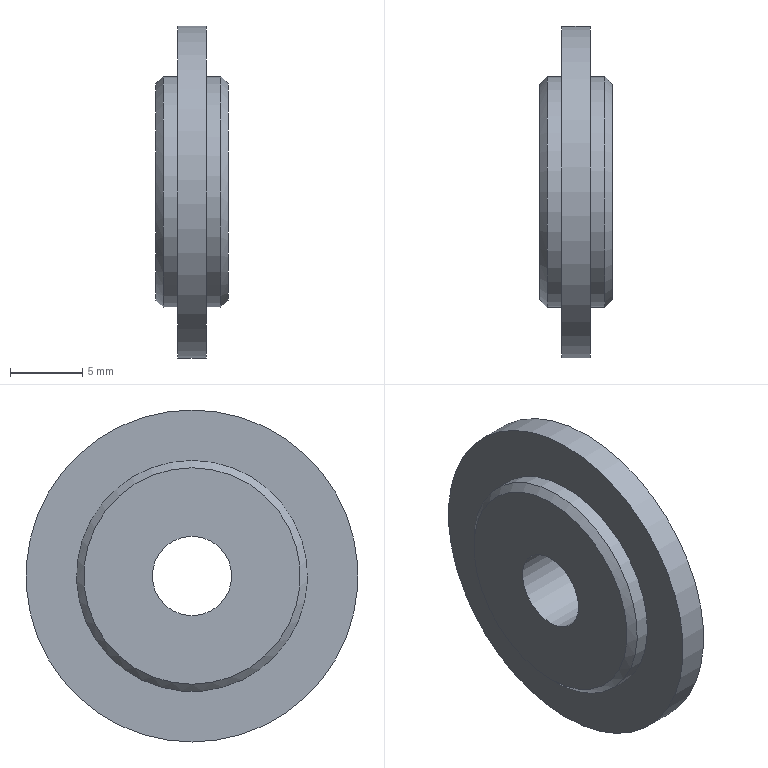Component | NX | MIDDLE_SPACER | 1 solid | 10 faces | box 5 x 23 x 23 mm | volume 1303 mm3 | cylinder 4 | plane 4 | cone 2 | commonest cylinder face diameters 16 x2 23 x1 5.5 x1
STEP:
#1=CARTESIAN_POINT('',(0.,0.,0.));
#2=DIRECTION('',(0.,0.,1.));
#3=DIRECTION('',(1.,0.,0.));
#4=AXIS2_PLACEMENT_3D('',#1,#2,#3);
#5=CARTESIAN_POINT('',(95.166,163.398,160.15));
#6=VERTEX_POINT('',#5);
#7=CARTESIAN_POINT('',(95.166,163.398,152.15));
#8=DIRECTION('',(-1.,0.,0.));
#9=DIRECTION('',(0.,0.,1.));
#10=AXIS2_PLACEMENT_3D('',#7,#8,#9);
#11=CIRCLE('',#10,8.);
#12=CARTESIAN_POINT('',(94.166,163.398,152.15));
#13=DIRECTION('',(1.,0.,0.));
#14=DIRECTION('',(0.,0.,-1.));
#15=AXIS2_PLACEMENT_3D('',#12,#13,#14);
#16=CYLINDRICAL_SURFACE('',#15,8.);
#17=CARTESIAN_POINT('',(9.425,1.));
#18=DIRECTION('',(-1.,0.));
#19=VECTOR('',#18,1.);
#20=LINE('',#17,#19);
#21=(GEOMETRIC_REPRESENTATION_CONTEXT(2)PARAMETRIC_REPRESENTATION_CONTEXT()REPRESENTATION_CONTEXT('',''));
#22=DEFINITIONAL_REPRESENTATION('',(#20),#21);
#23=PCURVE('',#16,#22);
#24=CARTESIAN_POINT('',(95.166,163.398,152.15));
#25=DIRECTION('',(-1.,0.,0.));
#26=DIRECTION('',(0.,0.,1.));
#27=AXIS2_PLACEMENT_3D('',#24,#25,#26);
#28=CONICAL_SURFACE('',#27,8.,0.7854);
#29=CARTESIAN_POINT('',(0.,0.));
#30=DIRECTION('',(1.,0.));
#31=VECTOR('',#30,1.);
#32=LINE('',#29,#31);
#33=(GEOMETRIC_REPRESENTATION_CONTEXT(2)PARAMETRIC_REPRESENTATION_CONTEXT()REPRESENTATION_CONTEXT('',''));
#34=DEFINITIONAL_REPRESENTATION('',(#32),#33);
#35=PCURVE('',#28,#34);
#36=SURFACE_CURVE('',#11,(#23,#35),.PCURVE_S1.);
#37=EDGE_CURVE('',#6,#6,#36,.T.);
#38=ORIENTED_EDGE('',*,*,#37,.T.);
#39=CARTESIAN_POINT('',(94.166,163.398,160.15));
#40=VERTEX_POINT('',#39);
#41=CARTESIAN_POINT('',(94.166,163.398,160.15));
#42=CARTESIAN_POINT('',(95.166,163.398,160.15));
#43=B_SPLINE_CURVE_WITH_KNOTS('',1,(#41,#42),.UNSPECIFIED.,.F.,.F.,(2,2),(0.,1.),.PIECEWISE_BEZIER_KNOTS.);
#44=CARTESIAN_POINT('',(3.142,0.));
#45=DIRECTION('',(0.,1.));
#46=VECTOR('',#45,1.);
#47=LINE('',#44,#46);
#48=(GEOMETRIC_REPRESENTATION_CONTEXT(2)PARAMETRIC_REPRESENTATION_CONTEXT()REPRESENTATION_CONTEXT('',''));
#49=DEFINITIONAL_REPRESENTATION('',(#47),#48);
#50=PCURVE('',#16,#49);
#51=CARTESIAN_POINT('',(9.425,0.));
#52=DIRECTION('',(0.,1.));
#53=VECTOR('',#52,1.);
#54=LINE('',#51,#53);
#55=(GEOMETRIC_REPRESENTATION_CONTEXT(2)PARAMETRIC_REPRESENTATION_CONTEXT()REPRESENTATION_CONTEXT('',''));
#56=DEFINITIONAL_REPRESENTATION('',(#54),#55);
#57=PCURVE('',#16,#56);
#58=SEAM_CURVE('',#43,(#50,#57),.PCURVE_S1.);
#59=EDGE_CURVE('',#40,#6,#58,.T.);
#60=ORIENTED_EDGE('',*,*,#59,.F.);
#61=CARTESIAN_POINT('',(94.166,163.398,152.15));
#62=DIRECTION('',(-1.,0.,0.));
#63=DIRECTION('',(0.,0.,1.));
#64=AXIS2_PLACEMENT_3D('',#61,#62,#63);
#65=CIRCLE('',#64,8.);
#66=CARTESIAN_POINT('',(9.425,0.));
#67=DIRECTION('',(-1.,0.));
#68=VECTOR('',#67,1.);
#69=LINE('',#66,#68);
#70=(GEOMETRIC_REPRESENTATION_CONTEXT(2)PARAMETRIC_REPRESENTATION_CONTEXT()REPRESENTATION_CONTEXT('',''));
#71=DEFINITIONAL_REPRESENTATION('',(#69),#70);
#72=PCURVE('',#16,#71);
#73=CARTESIAN_POINT('',(94.166,163.398,152.15));
#74=DIRECTION('',(-1.,0.,0.));
#75=DIRECTION('',(0.,0.,1.));
#76=AXIS2_PLACEMENT_3D('',#73,#74,#75);
#77=PLANE('',#76);
#78=CARTESIAN_POINT('',(0.,0.));
#79=DIRECTION('',(1.,0.));
#80=AXIS2_PLACEMENT_2D('',#78,#79);
#81=CIRCLE('',#80,8.);
#82=(GEOMETRIC_REPRESENTATION_CONTEXT(2)PARAMETRIC_REPRESENTATION_CONTEXT()REPRESENTATION_CONTEXT('',''));
#83=DEFINITIONAL_REPRESENTATION('',(#81),#82);
#84=PCURVE('',#77,#83);
#85=SURFACE_CURVE('',#65,(#72,#84),.PCURVE_S1.);
#86=EDGE_CURVE('',#40,#40,#85,.T.);
#87=ORIENTED_EDGE('',*,*,#86,.F.);
#88=ORIENTED_EDGE('',*,*,#59,.T.);
#89=EDGE_LOOP('',(#38,#60,#87,#88));
#90=FACE_BOUND('',#89,.T.);
#91=ADVANCED_FACE('',(#90),#16,.T.);
#92=CARTESIAN_POINT('',(95.666,163.398,159.65));
#93=VERTEX_POINT('',#92);
#94=CARTESIAN_POINT('',(95.666,163.398,152.15));
#95=DIRECTION('',(1.,0.,0.));
#96=DIRECTION('',(0.,0.,1.));
#97=AXIS2_PLACEMENT_3D('',#94,#95,#96);
#98=CIRCLE('',#97,7.5);
#99=CARTESIAN_POINT('',(95.666,163.398,152.15));
#100=DIRECTION('',(-1.,0.,0.));
#101=DIRECTION('',(0.,0.,1.));
#102=AXIS2_PLACEMENT_3D('',#99,#100,#101);
#103=PLANE('',#102);
#104=CARTESIAN_POINT('',(7.5,0.));
#105=CARTESIAN_POINT('',(7.5,-12.99));
#106=CARTESIAN_POINT('',(-3.75,-6.495));
#107=CARTESIAN_POINT('',(-15.,-0.));
#108=CARTESIAN_POINT('',(-3.75,6.495));
#109=CARTESIAN_POINT('',(7.5,12.99));
#110=CARTESIAN_POINT('',(7.5,0.));
#111=(BOUNDED_CURVE()B_SPLINE_CURVE(2,(#104,#105,#106,#107,#108,#109,#110),.UNSPECIFIED.,.T.,.F.)B_SPLINE_CURVE_WITH_KNOTS((1,2,2,2,2,1),(-2.094,0.,2.094,4.189,6.283,8.378),.UNSPECIFIED.)CURVE()GEOMETRIC_REPRESENTATION_ITEM()RATIONAL_B_SPLINE_CURVE((1.,0.5,1.,0.5,1.,0.5,1.))REPRESENTATION_ITEM(''));
#112=(GEOMETRIC_REPRESENTATION_CONTEXT(2)PARAMETRIC_REPRESENTATION_CONTEXT()REPRESENTATION_CONTEXT('',''));
#113=DEFINITIONAL_REPRESENTATION('',(#111),#112);
#114=PCURVE('',#103,#113);
#115=CARTESIAN_POINT('',(6.283,-0.5));
#116=DIRECTION('',(-1.,0.));
#117=VECTOR('',#116,1.);
#118=LINE('',#115,#117);
#119=(GEOMETRIC_REPRESENTATION_CONTEXT(2)PARAMETRIC_REPRESENTATION_CONTEXT()REPRESENTATION_CONTEXT('',''));
#120=DEFINITIONAL_REPRESENTATION('',(#118),#119);
#121=PCURVE('',#28,#120);
#122=SURFACE_CURVE('',#98,(#114,#121),.PCURVE_S1.);
#123=EDGE_CURVE('',#93,#93,#122,.T.);
#124=ORIENTED_EDGE('',*,*,#123,.T.);
#125=EDGE_LOOP('',(#124));
#126=FACE_BOUND('',#125,.T.);
#127=CARTESIAN_POINT('',(95.666,163.398,154.9));
#128=VERTEX_POINT('',#127);
#129=CARTESIAN_POINT('',(95.666,163.398,152.15));
#130=DIRECTION('',(-1.,0.,0.));
#131=DIRECTION('',(0.,0.,1.));
#132=AXIS2_PLACEMENT_3D('',#129,#130,#131);
#133=CIRCLE('',#132,2.75);
#134=CARTESIAN_POINT('',(0.,0.));
#135=DIRECTION('',(1.,0.));
#136=AXIS2_PLACEMENT_2D('',#134,#135);
#137=CIRCLE('',#136,2.75);
#138=(GEOMETRIC_REPRESENTATION_CONTEXT(2)PARAMETRIC_REPRESENTATION_CONTEXT()REPRESENTATION_CONTEXT('',''));
#139=DEFINITIONAL_REPRESENTATION('',(#137),#138);
#140=PCURVE('',#103,#139);
#141=CARTESIAN_POINT('',(112.666,163.398,152.15));
#142=DIRECTION('',(-1.,0.,0.));
#143=DIRECTION('',(0.,0.,1.));
#144=AXIS2_PLACEMENT_3D('',#141,#142,#143);
#145=CYLINDRICAL_SURFACE('',#144,2.75);
#146=CARTESIAN_POINT('',(0.,17.));
#147=DIRECTION('',(1.,0.));
#148=VECTOR('',#147,1.);
#149=LINE('',#146,#148);
#150=(GEOMETRIC_REPRESENTATION_CONTEXT(2)PARAMETRIC_REPRESENTATION_CONTEXT()REPRESENTATION_CONTEXT('',''));
#151=DEFINITIONAL_REPRESENTATION('',(#149),#150);
#152=PCURVE('',#145,#151);
#153=SURFACE_CURVE('',#133,(#140,#152),.PCURVE_S1.);
#154=EDGE_CURVE('',#128,#128,#153,.T.);
#155=ORIENTED_EDGE('',*,*,#154,.T.);
#156=EDGE_LOOP('',(#155));
#157=FACE_BOUND('',#156,.T.);
#158=ADVANCED_FACE('',(#126,#157),#103,.F.);
#159=CARTESIAN_POINT('',(92.166,163.398,163.65));
#160=VERTEX_POINT('',#159);
#161=CARTESIAN_POINT('',(92.166,163.398,152.15));
#162=DIRECTION('',(-1.,0.,0.));
#163=DIRECTION('',(0.,0.,1.));
#164=AXIS2_PLACEMENT_3D('',#161,#162,#163);
#165=CIRCLE('',#164,11.5);
#166=CARTESIAN_POINT('',(92.166,163.398,152.15));
#167=DIRECTION('',(1.,0.,0.));
#168=DIRECTION('',(0.,0.,-1.));
#169=AXIS2_PLACEMENT_3D('',#166,#167,#168);
#170=CYLINDRICAL_SURFACE('',#169,11.5);
#171=CARTESIAN_POINT('',(9.425,0.));
#172=DIRECTION('',(-1.,0.));
#173=VECTOR('',#172,1.);
#174=LINE('',#171,#173);
#175=(GEOMETRIC_REPRESENTATION_CONTEXT(2)PARAMETRIC_REPRESENTATION_CONTEXT()REPRESENTATION_CONTEXT('',''));
#176=DEFINITIONAL_REPRESENTATION('',(#174),#175);
#177=PCURVE('',#170,#176);
#178=CARTESIAN_POINT('',(92.166,163.398,152.15));
#179=DIRECTION('',(-1.,0.,0.));
#180=DIRECTION('',(0.,0.,1.));
#181=AXIS2_PLACEMENT_3D('',#178,#179,#180);
#182=PLANE('',#181);
#183=CARTESIAN_POINT('',(0.,0.));
#184=DIRECTION('',(1.,0.));
#185=AXIS2_PLACEMENT_2D('',#183,#184);
#186=CIRCLE('',#185,11.5);
#187=(GEOMETRIC_REPRESENTATION_CONTEXT(2)PARAMETRIC_REPRESENTATION_CONTEXT()REPRESENTATION_CONTEXT('',''));
#188=DEFINITIONAL_REPRESENTATION('',(#186),#187);
#189=PCURVE('',#182,#188);
#190=SURFACE_CURVE('',#165,(#177,#189),.PCURVE_S1.);
#191=EDGE_CURVE('',#160,#160,#190,.T.);
#192=ORIENTED_EDGE('',*,*,#191,.F.);
#193=CARTESIAN_POINT('',(94.166,163.398,163.65));
#194=VERTEX_POINT('',#193);
#195=CARTESIAN_POINT('',(92.166,163.398,163.65));
#196=CARTESIAN_POINT('',(94.166,163.398,163.65));
#197=B_SPLINE_CURVE_WITH_KNOTS('',1,(#195,#196),.UNSPECIFIED.,.F.,.F.,(2,2),(0.,2.),.PIECEWISE_BEZIER_KNOTS.);
#198=CARTESIAN_POINT('',(9.425,0.));
#199=DIRECTION('',(0.,1.));
#200=VECTOR('',#199,1.);
#201=LINE('',#198,#200);
#202=(GEOMETRIC_REPRESENTATION_CONTEXT(2)PARAMETRIC_REPRESENTATION_CONTEXT()REPRESENTATION_CONTEXT('',''));
#203=DEFINITIONAL_REPRESENTATION('',(#201),#202);
#204=PCURVE('',#170,#203);
#205=CARTESIAN_POINT('',(3.142,0.));
#206=DIRECTION('',(0.,1.));
#207=VECTOR('',#206,1.);
#208=LINE('',#205,#207);
#209=(GEOMETRIC_REPRESENTATION_CONTEXT(2)PARAMETRIC_REPRESENTATION_CONTEXT()REPRESENTATION_CONTEXT('',''));
#210=DEFINITIONAL_REPRESENTATION('',(#208),#209);
#211=PCURVE('',#170,#210);
#212=SEAM_CURVE('',#197,(#204,#211),.PCURVE_S1.);
#213=EDGE_CURVE('',#160,#194,#212,.T.);
#214=ORIENTED_EDGE('',*,*,#213,.T.);
#215=CARTESIAN_POINT('',(94.166,163.398,152.15));
#216=DIRECTION('',(-1.,0.,0.));
#217=DIRECTION('',(0.,0.,1.));
#218=AXIS2_PLACEMENT_3D('',#215,#216,#217);
#219=CIRCLE('',#218,11.5);
#220=CARTESIAN_POINT('',(9.425,2.));
#221=DIRECTION('',(-1.,0.));
#222=VECTOR('',#221,1.);
#223=LINE('',#220,#222);
#224=(GEOMETRIC_REPRESENTATION_CONTEXT(2)PARAMETRIC_REPRESENTATION_CONTEXT()REPRESENTATION_CONTEXT('',''));
#225=DEFINITIONAL_REPRESENTATION('',(#223),#224);
#226=PCURVE('',#170,#225);
#227=CARTESIAN_POINT('',(0.,0.));
#228=DIRECTION('',(1.,0.));
#229=AXIS2_PLACEMENT_2D('',#227,#228);
#230=CIRCLE('',#229,11.5);
#231=(GEOMETRIC_REPRESENTATION_CONTEXT(2)PARAMETRIC_REPRESENTATION_CONTEXT()REPRESENTATION_CONTEXT('',''));
#232=DEFINITIONAL_REPRESENTATION('',(#230),#231);
#233=PCURVE('',#77,#232);
#234=SURFACE_CURVE('',#219,(#226,#233),.PCURVE_S1.);
#235=EDGE_CURVE('',#194,#194,#234,.T.);
#236=ORIENTED_EDGE('',*,*,#235,.T.);
#237=ORIENTED_EDGE('',*,*,#213,.F.);
#238=EDGE_LOOP('',(#192,#214,#236,#237));
#239=FACE_BOUND('',#238,.T.);
#240=ADVANCED_FACE('',(#239),#170,.T.);
#241=CARTESIAN_POINT('',(92.166,163.398,160.15));
#242=VERTEX_POINT('',#241);
#243=CARTESIAN_POINT('',(92.166,163.398,152.15));
#244=DIRECTION('',(-1.,0.,0.));
#245=DIRECTION('',(0.,0.,1.));
#246=AXIS2_PLACEMENT_3D('',#243,#244,#245);
#247=CIRCLE('',#246,8.);
#248=CARTESIAN_POINT('',(0.,0.));
#249=DIRECTION('',(1.,0.));
#250=AXIS2_PLACEMENT_2D('',#248,#249);
#251=CIRCLE('',#250,8.);
#252=(GEOMETRIC_REPRESENTATION_CONTEXT(2)PARAMETRIC_REPRESENTATION_CONTEXT()REPRESENTATION_CONTEXT('',''));
#253=DEFINITIONAL_REPRESENTATION('',(#251),#252);
#254=PCURVE('',#182,#253);
#255=CARTESIAN_POINT('',(90.666,163.398,152.15));
#256=DIRECTION('',(1.,0.,0.));
#257=DIRECTION('',(0.,0.,-1.));
#258=AXIS2_PLACEMENT_3D('',#255,#256,#257);
#259=CYLINDRICAL_SURFACE('',#258,8.);
#260=CARTESIAN_POINT('',(9.425,1.5));
#261=DIRECTION('',(-1.,0.));
#262=VECTOR('',#261,1.);
#263=LINE('',#260,#262);
#264=(GEOMETRIC_REPRESENTATION_CONTEXT(2)PARAMETRIC_REPRESENTATION_CONTEXT()REPRESENTATION_CONTEXT('',''));
#265=DEFINITIONAL_REPRESENTATION('',(#263),#264);
#266=PCURVE('',#259,#265);
#267=SURFACE_CURVE('',#247,(#254,#266),.PCURVE_S1.);
#268=EDGE_CURVE('',#242,#242,#267,.T.);
#269=ORIENTED_EDGE('',*,*,#268,.F.);
#270=EDGE_LOOP('',(#269));
#271=FACE_BOUND('',#270,.T.);
#272=ORIENTED_EDGE('',*,*,#191,.T.);
#273=EDGE_LOOP('',(#272));
#274=FACE_BOUND('',#273,.T.);
#275=ADVANCED_FACE('',(#271,#274),#182,.T.);
#276=ORIENTED_EDGE('',*,*,#86,.T.);
#277=EDGE_LOOP('',(#276));
#278=FACE_BOUND('',#277,.T.);
#279=ORIENTED_EDGE('',*,*,#235,.F.);
#280=EDGE_LOOP('',(#279));
#281=FACE_BOUND('',#280,.T.);
#282=ADVANCED_FACE('',(#278,#281),#77,.F.);
#283=CARTESIAN_POINT('',(91.166,163.398,160.15));
#284=VERTEX_POINT('',#283);
#285=CARTESIAN_POINT('',(91.166,163.398,152.15));
#286=DIRECTION('',(1.,0.,0.));
#287=DIRECTION('',(0.,0.,1.));
#288=AXIS2_PLACEMENT_3D('',#285,#286,#287);
#289=CIRCLE('',#288,8.);
#290=CARTESIAN_POINT('',(3.142,0.5));
#291=DIRECTION('',(1.,0.));
#292=VECTOR('',#291,1.);
#293=LINE('',#290,#292);
#294=(GEOMETRIC_REPRESENTATION_CONTEXT(2)PARAMETRIC_REPRESENTATION_CONTEXT()REPRESENTATION_CONTEXT('',''));
#295=DEFINITIONAL_REPRESENTATION('',(#293),#294);
#296=PCURVE('',#259,#295);
#297=CARTESIAN_POINT('',(90.666,163.398,152.15));
#298=DIRECTION('',(1.,0.,0.));
#299=DIRECTION('',(0.,0.,-1.));
#300=AXIS2_PLACEMENT_3D('',#297,#298,#299);
#301=CONICAL_SURFACE('',#300,7.5,0.7854);
#302=CARTESIAN_POINT('',(3.142,0.5));
#303=DIRECTION('',(1.,0.));
#304=VECTOR('',#303,1.);
#305=LINE('',#302,#304);
#306=(GEOMETRIC_REPRESENTATION_CONTEXT(2)PARAMETRIC_REPRESENTATION_CONTEXT()REPRESENTATION_CONTEXT('',''));
#307=DEFINITIONAL_REPRESENTATION('',(#305),#306);
#308=PCURVE('',#301,#307);
#309=SURFACE_CURVE('',#289,(#296,#308),.PCURVE_S1.);
#310=EDGE_CURVE('',#284,#284,#309,.T.);
#311=ORIENTED_EDGE('',*,*,#310,.T.);
#312=CARTESIAN_POINT('',(91.166,163.398,160.15));
#313=CARTESIAN_POINT('',(92.166,163.398,160.15));
#314=B_SPLINE_CURVE_WITH_KNOTS('',1,(#312,#313),.UNSPECIFIED.,.F.,.F.,(2,2),(0.5,1.5),.PIECEWISE_BEZIER_KNOTS.);
#315=CARTESIAN_POINT('',(9.425,0.));
#316=DIRECTION('',(0.,1.));
#317=VECTOR('',#316,1.);
#318=LINE('',#315,#317);
#319=(GEOMETRIC_REPRESENTATION_CONTEXT(2)PARAMETRIC_REPRESENTATION_CONTEXT()REPRESENTATION_CONTEXT('',''));
#320=DEFINITIONAL_REPRESENTATION('',(#318),#319);
#321=PCURVE('',#259,#320);
#322=CARTESIAN_POINT('',(3.142,0.));
#323=DIRECTION('',(0.,1.));
#324=VECTOR('',#323,1.);
#325=LINE('',#322,#324);
#326=(GEOMETRIC_REPRESENTATION_CONTEXT(2)PARAMETRIC_REPRESENTATION_CONTEXT()REPRESENTATION_CONTEXT('',''));
#327=DEFINITIONAL_REPRESENTATION('',(#325),#326);
#328=PCURVE('',#259,#327);
#329=SEAM_CURVE('',#314,(#321,#328),.PCURVE_S1.);
#330=EDGE_CURVE('',#284,#242,#329,.T.);
#331=ORIENTED_EDGE('',*,*,#330,.T.);
#332=ORIENTED_EDGE('',*,*,#268,.T.);
#333=ORIENTED_EDGE('',*,*,#330,.F.);
#334=EDGE_LOOP('',(#311,#331,#332,#333));
#335=FACE_BOUND('',#334,.T.);
#336=ADVANCED_FACE('',(#335),#259,.T.);
#337=CARTESIAN_POINT('',(90.666,163.398,159.65));
#338=VERTEX_POINT('',#337);
#339=CARTESIAN_POINT('',(90.666,163.398,152.15));
#340=DIRECTION('',(-1.,0.,0.));
#341=DIRECTION('',(0.,0.,1.));
#342=AXIS2_PLACEMENT_3D('',#339,#340,#341);
#343=CIRCLE('',#342,7.5);
#344=CARTESIAN_POINT('',(90.666,163.398,152.15));
#345=DIRECTION('',(-1.,0.,0.));
#346=DIRECTION('',(0.,0.,1.));
#347=AXIS2_PLACEMENT_3D('',#344,#345,#346);
#348=PLANE('',#347);
#349=CARTESIAN_POINT('',(0.,0.));
#350=DIRECTION('',(1.,0.));
#351=AXIS2_PLACEMENT_2D('',#349,#350);
#352=CIRCLE('',#351,7.5);
#353=(GEOMETRIC_REPRESENTATION_CONTEXT(2)PARAMETRIC_REPRESENTATION_CONTEXT()REPRESENTATION_CONTEXT('',''));
#354=DEFINITIONAL_REPRESENTATION('',(#352),#353);
#355=PCURVE('',#348,#354);
#356=CARTESIAN_POINT('',(9.425,0.));
#357=DIRECTION('',(-1.,0.));
#358=VECTOR('',#357,1.);
#359=LINE('',#356,#358);
#360=(GEOMETRIC_REPRESENTATION_CONTEXT(2)PARAMETRIC_REPRESENTATION_CONTEXT()REPRESENTATION_CONTEXT('',''));
#361=DEFINITIONAL_REPRESENTATION('',(#359),#360);
#362=PCURVE('',#301,#361);
#363=SURFACE_CURVE('',#343,(#355,#362),.PCURVE_S1.);
#364=EDGE_CURVE('',#338,#338,#363,.T.);
#365=ORIENTED_EDGE('',*,*,#364,.T.);
#366=EDGE_LOOP('',(#365));
#367=FACE_BOUND('',#366,.T.);
#368=CARTESIAN_POINT('',(90.666,163.398,154.9));
#369=VERTEX_POINT('',#368);
#370=CARTESIAN_POINT('',(90.666,163.398,152.15));
#371=DIRECTION('',(-1.,0.,0.));
#372=DIRECTION('',(0.,0.,1.));
#373=AXIS2_PLACEMENT_3D('',#370,#371,#372);
#374=CIRCLE('',#373,2.75);
#375=CARTESIAN_POINT('',(0.,0.));
#376=DIRECTION('',(1.,0.));
#377=AXIS2_PLACEMENT_2D('',#375,#376);
#378=CIRCLE('',#377,2.75);
#379=(GEOMETRIC_REPRESENTATION_CONTEXT(2)PARAMETRIC_REPRESENTATION_CONTEXT()REPRESENTATION_CONTEXT('',''));
#380=DEFINITIONAL_REPRESENTATION('',(#378),#379);
#381=PCURVE('',#348,#380);
#382=CARTESIAN_POINT('',(0.,22.));
#383=DIRECTION('',(1.,0.));
#384=VECTOR('',#383,1.);
#385=LINE('',#382,#384);
#386=(GEOMETRIC_REPRESENTATION_CONTEXT(2)PARAMETRIC_REPRESENTATION_CONTEXT()REPRESENTATION_CONTEXT('',''));
#387=DEFINITIONAL_REPRESENTATION('',(#385),#386);
#388=PCURVE('',#145,#387);
#389=SURFACE_CURVE('',#374,(#381,#388),.PCURVE_S1.);
#390=EDGE_CURVE('',#369,#369,#389,.T.);
#391=ORIENTED_EDGE('',*,*,#390,.F.);
#392=EDGE_LOOP('',(#391));
#393=FACE_BOUND('',#392,.T.);
#394=ADVANCED_FACE('',(#367,#393),#348,.T.);
#395=ORIENTED_EDGE('',*,*,#390,.F.);
#396=CARTESIAN_POINT('',(95.666,163.398,154.9));
#397=CARTESIAN_POINT('',(90.666,163.398,154.9));
#398=B_SPLINE_CURVE_WITH_KNOTS('',1,(#396,#397),.UNSPECIFIED.,.F.,.F.,(2,2),(17.,22.),.PIECEWISE_BEZIER_KNOTS.);
#399=CARTESIAN_POINT('',(0.,0.));
#400=DIRECTION('',(0.,1.));
#401=VECTOR('',#400,1.);
#402=LINE('',#399,#401);
#403=(GEOMETRIC_REPRESENTATION_CONTEXT(2)PARAMETRIC_REPRESENTATION_CONTEXT()REPRESENTATION_CONTEXT('',''));
#404=DEFINITIONAL_REPRESENTATION('',(#402),#403);
#405=PCURVE('',#145,#404);
#406=CARTESIAN_POINT('',(6.283,0.));
#407=DIRECTION('',(0.,1.));
#408=VECTOR('',#407,1.);
#409=LINE('',#406,#408);
#410=(GEOMETRIC_REPRESENTATION_CONTEXT(2)PARAMETRIC_REPRESENTATION_CONTEXT()REPRESENTATION_CONTEXT('',''));
#411=DEFINITIONAL_REPRESENTATION('',(#409),#410);
#412=PCURVE('',#145,#411);
#413=SEAM_CURVE('',#398,(#405,#412),.PCURVE_S1.);
#414=EDGE_CURVE('',#128,#369,#413,.T.);
#415=ORIENTED_EDGE('',*,*,#414,.F.);
#416=ORIENTED_EDGE('',*,*,#154,.T.);
#417=ORIENTED_EDGE('',*,*,#414,.T.);
#418=EDGE_LOOP('',(#395,#415,#416,#417));
#419=FACE_BOUND('',#418,.F.);
#420=ADVANCED_FACE('',(#419),#145,.F.);
#421=ORIENTED_EDGE('',*,*,#123,.F.);
#422=CARTESIAN_POINT('',(95.666,163.398,159.65));
#423=CARTESIAN_POINT('',(95.166,163.398,160.15));
#424=B_SPLINE_CURVE_WITH_KNOTS('',1,(#422,#423),.UNSPECIFIED.,.F.,.F.,(2,2),(-0.7071,0.),.PIECEWISE_BEZIER_KNOTS.);
#425=CARTESIAN_POINT('',(6.283,0.));
#426=DIRECTION('',(0.,1.));
#427=VECTOR('',#426,1.);
#428=LINE('',#425,#427);
#429=(GEOMETRIC_REPRESENTATION_CONTEXT(2)PARAMETRIC_REPRESENTATION_CONTEXT()REPRESENTATION_CONTEXT('',''));
#430=DEFINITIONAL_REPRESENTATION('',(#428),#429);
#431=PCURVE('',#28,#430);
#432=CARTESIAN_POINT('',(0.,0.));
#433=DIRECTION('',(0.,1.));
#434=VECTOR('',#433,1.);
#435=LINE('',#432,#434);
#436=(GEOMETRIC_REPRESENTATION_CONTEXT(2)PARAMETRIC_REPRESENTATION_CONTEXT()REPRESENTATION_CONTEXT('',''));
#437=DEFINITIONAL_REPRESENTATION('',(#435),#436);
#438=PCURVE('',#28,#437);
#439=SEAM_CURVE('',#424,(#431,#438),.PCURVE_S1.);
#440=EDGE_CURVE('',#93,#6,#439,.T.);
#441=ORIENTED_EDGE('',*,*,#440,.T.);
#442=ORIENTED_EDGE('',*,*,#37,.F.);
#443=ORIENTED_EDGE('',*,*,#440,.F.);
#444=EDGE_LOOP('',(#421,#441,#442,#443));
#445=FACE_BOUND('',#444,.T.);
#446=ADVANCED_FACE('',(#445),#28,.T.);
#447=ORIENTED_EDGE('',*,*,#310,.F.);
#448=CARTESIAN_POINT('',(90.666,163.398,159.65));
#449=CARTESIAN_POINT('',(91.166,163.398,160.15));
#450=B_SPLINE_CURVE_WITH_KNOTS('',1,(#448,#449),.UNSPECIFIED.,.F.,.F.,(2,2),(0.,0.7071),.PIECEWISE_BEZIER_KNOTS.);
#451=CARTESIAN_POINT('',(3.142,0.));
#452=DIRECTION('',(0.,1.));
#453=VECTOR('',#452,1.);
#454=LINE('',#451,#453);
#455=(GEOMETRIC_REPRESENTATION_CONTEXT(2)PARAMETRIC_REPRESENTATION_CONTEXT()REPRESENTATION_CONTEXT('',''));
#456=DEFINITIONAL_REPRESENTATION('',(#454),#455);
#457=PCURVE('',#301,#456);
#458=CARTESIAN_POINT('',(9.425,0.));
#459=DIRECTION('',(0.,1.));
#460=VECTOR('',#459,1.);
#461=LINE('',#458,#460);
#462=(GEOMETRIC_REPRESENTATION_CONTEXT(2)PARAMETRIC_REPRESENTATION_CONTEXT()REPRESENTATION_CONTEXT('',''));
#463=DEFINITIONAL_REPRESENTATION('',(#461),#462);
#464=PCURVE('',#301,#463);
#465=SEAM_CURVE('',#450,(#457,#464),.PCURVE_S1.);
#466=EDGE_CURVE('',#338,#284,#465,.T.);
#467=ORIENTED_EDGE('',*,*,#466,.F.);
#468=ORIENTED_EDGE('',*,*,#364,.F.);
#469=ORIENTED_EDGE('',*,*,#466,.T.);
#470=EDGE_LOOP('',(#447,#467,#468,#469));
#471=FACE_BOUND('',#470,.T.);
#472=ADVANCED_FACE('',(#471),#301,.T.);
#473=CLOSED_SHELL('',(#91,#158,#240,#275,#282,#336,#394,#420,#446,#472));
#474=MANIFOLD_SOLID_BREP('',#473);
#475=(LENGTH_UNIT()NAMED_UNIT(*)SI_UNIT(.MILLI.,.METRE.));
#476=UNCERTAINTY_MEASURE_WITH_UNIT(LENGTH_MEASURE(0.00001),#475,'','');
#477=(NAMED_UNIT(*)PLANE_ANGLE_UNIT()SI_UNIT($,.RADIAN.));
#478=(NAMED_UNIT(*)SI_UNIT($,.STERADIAN.)SOLID_ANGLE_UNIT());
#479=(GEOMETRIC_REPRESENTATION_CONTEXT(3)GLOBAL_UNCERTAINTY_ASSIGNED_CONTEXT((#476))GLOBAL_UNIT_ASSIGNED_CONTEXT((#475,#477,#478))REPRESENTATION_CONTEXT('',''));
#480=ADVANCED_BREP_SHAPE_REPRESENTATION('',(#4,#474),#479);